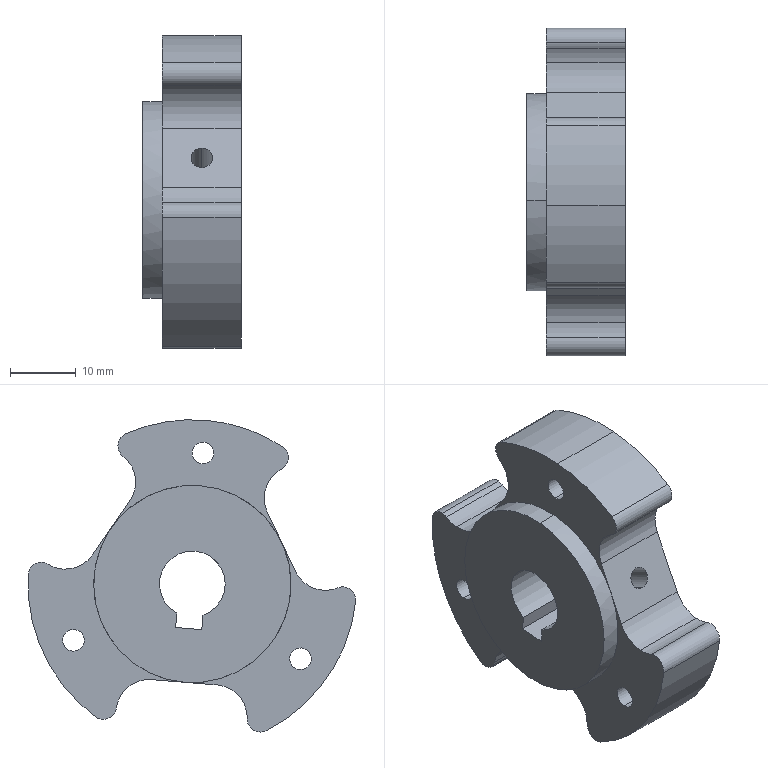Component | SolidWorks | 2018SOLIDWORKS1000000024-1 | 1 solid | 48 faces | box 15 x 49.87 x 47.54 mm | volume 17417 mm3 | cylinder 34 | plane 11 | cone 3 | commonest cylinder face diameters 3.3 x10 10 x10 4 x8 50 x4 30 x2 | material 6061 Alloy
build123d program:
from build123d import *

# Parameters (mm, degrees)
SKETCH1_R           = 25
SKETCH1_R_2         = 8.5
BOSS_EXTRUDE1_DEPTH = 12
M4_TAPPED_HOLE1_D   = 3.3
CIRPATTERN1_COUNT   = 3
SKETCH8_R           = 8.5
SKETCH8_R_2         = 5
BOSS_EXTRUDE2_DEPTH = 12
BOSS_EXTRUDE3_START = 3
SKETCH10_R          = 15
SKETCH10_R_2        = 5
BOSS_EXTRUDE3_DEPTH = 3
SKETCH11_W          = 4
SKETCH11_H          = 4
CUT_EXTRUDE4_DEPTH  = 39.406
SKETCH13_W          = 25
SKETCH13_H          = 20
CUT_EXTRUDE5_DEPTH  = 38.336
CIRPATTERN2_COUNT   = 3
FILLET2_R           = 5
FILLET3_R           = 2
CIRPATTERN3_COUNT   = 2
CIRPATTERN3_ANGLE   = 120


with BuildPart() as part:
    # Sketch1 → Boss-Extrude1 (new body)
    with BuildSketch(Plane.XY):
        Circle(SKETCH1_R)
        Circle(SKETCH1_R_2, mode=Mode.SUBTRACT)
    extrude(amount=BOSS_EXTRUDE1_DEPTH)

    # M4 Tapped Hole1 (through all)
    with Locations(Plane(origin=(-27.806, 3.666, 0), x_dir=(1, 0, 0), z_dir=(0, 0, -1))):
        with Locations((7.806, 3.666)):
            m4_tapped_hole1 = Hole(M4_TAPPED_HOLE1_D / 2)

    # CirPattern1: M4 Tapped Hole1 ×3 about axis
    cirpattern1_axis = Axis((0, 0, 0), (0, 0, 1))
    for i in range(1, CIRPATTERN1_COUNT):
        add(m4_tapped_hole1.rotate(cirpattern1_axis, i * 360 / CIRPATTERN1_COUNT), mode=Mode.SUBTRACT)

    # Sketch8 → Boss-Extrude2 (add)
    with BuildSketch(Plane(origin=(0, 0, 0), x_dir=(-1, 0, 0), z_dir=(0, 0, -1))):
        Circle(SKETCH8_R)
        Circle(SKETCH8_R_2, mode=Mode.SUBTRACT)
    extrude(amount=-BOSS_EXTRUDE2_DEPTH)

    # Sketch10 → Boss-Extrude3 (add)
    with BuildSketch(Plane(origin=(0, 0, 0), x_dir=(-1, 0, 0), z_dir=(0, 0, -1)).offset(BOSS_EXTRUDE3_START)):
        with Locations(Location((0, 0, 0), (0, 0, 180))):
            Circle(SKETCH10_R)
        Circle(SKETCH10_R_2, mode=Mode.SUBTRACT)
    extrude(amount=-BOSS_EXTRUDE3_DEPTH)

    # Sketch11 → Cut-Extrude4 (cut, through all)
    with BuildSketch(Plane(origin=(0, 0, -3), x_dir=(-1, 0, 0), z_dir=(0, 0, -1))):
        with Locations((-4.8, 0)):
            Rectangle(SKETCH11_W, SKETCH11_H)
    extrude(amount=-CUT_EXTRUDE4_DEPTH, mode=Mode.SUBTRACT)

    # Sketch13 → Cut-Extrude5 (cut, through all)
    with BuildSketch(Plane(origin=(0, 0, 0), x_dir=(-1, 0, 0), z_dir=(0, 0, -1))):
        with Locations((-27.5, 0)):
            Rectangle(SKETCH13_W, SKETCH13_H)
    cut_extrude5 = extrude(amount=-CUT_EXTRUDE5_DEPTH, mode=Mode.SUBTRACT)

    # CirPattern2: Cut-Extrude5 ×3 about axis
    cirpattern2_axis = Axis((0, 0, 0), (0, 0, 1))
    for i in range(1, CIRPATTERN2_COUNT):
        add(cut_extrude5.rotate(cirpattern2_axis, i * 360 / CIRPATTERN2_COUNT), mode=Mode.SUBTRACT)

    # Fillet2
    fillet2_edges = [part.edges().sort_by_distance(p)[0] for p in [
        (1.16, -17.99, 6),
        (15, -10, 6),
        (15, 10, 6),
        (1.16, 17.99, 6),
        (-16.16, 7.99, 6),
        (-16.16, -7.99, 6),
    ]]
    fillet(fillet2_edges, radius=FILLET2_R)

    # Fillet3
    fillet3_edges = [part.edges().sort_by_distance(p)[0] for p in [
        (22.913, 10, 6),
        (22.913, -10, 6),
        (-2.796, -24.843, 6),
        (-20.117, -14.843, 6),
        (-20.117, 14.843, 6),
        (-2.796, 24.843, 6),
    ]]
    fillet(fillet3_edges, radius=FILLET3_R)

    # Sketch15 → M4 Tapped Hole2 (revolve, cut)
    with BuildSketch(Plane(origin=(15, 0, 6), x_dir=(0, 0, -1), z_dir=(0, 1, 0))):
        Polygon((0, 0), (0, 11.091), (1.65, 10.1), (1.65, 0), align=None)
    m4_tapped_hole2 = revolve(axis=Axis((21.35, 0, 6), (-1, 0, 0)), mode=Mode.SUBTRACT)

    # CirPattern3: M4 Tapped Hole2 ×2 about axis
    cirpattern3_axis = Axis((0, 0, 12), (0, 0, -1))
    for i in range(1, CIRPATTERN3_COUNT):
        add(m4_tapped_hole2.rotate(cirpattern3_axis, i * CIRPATTERN3_ANGLE / (CIRPATTERN3_COUNT - 1)), mode=Mode.SUBTRACT)


solid = part.part

# Placed as in the assembly
solid = solid.moved(Location((-11.284, -95.825, 207.018), (4.654, 90, 0)))